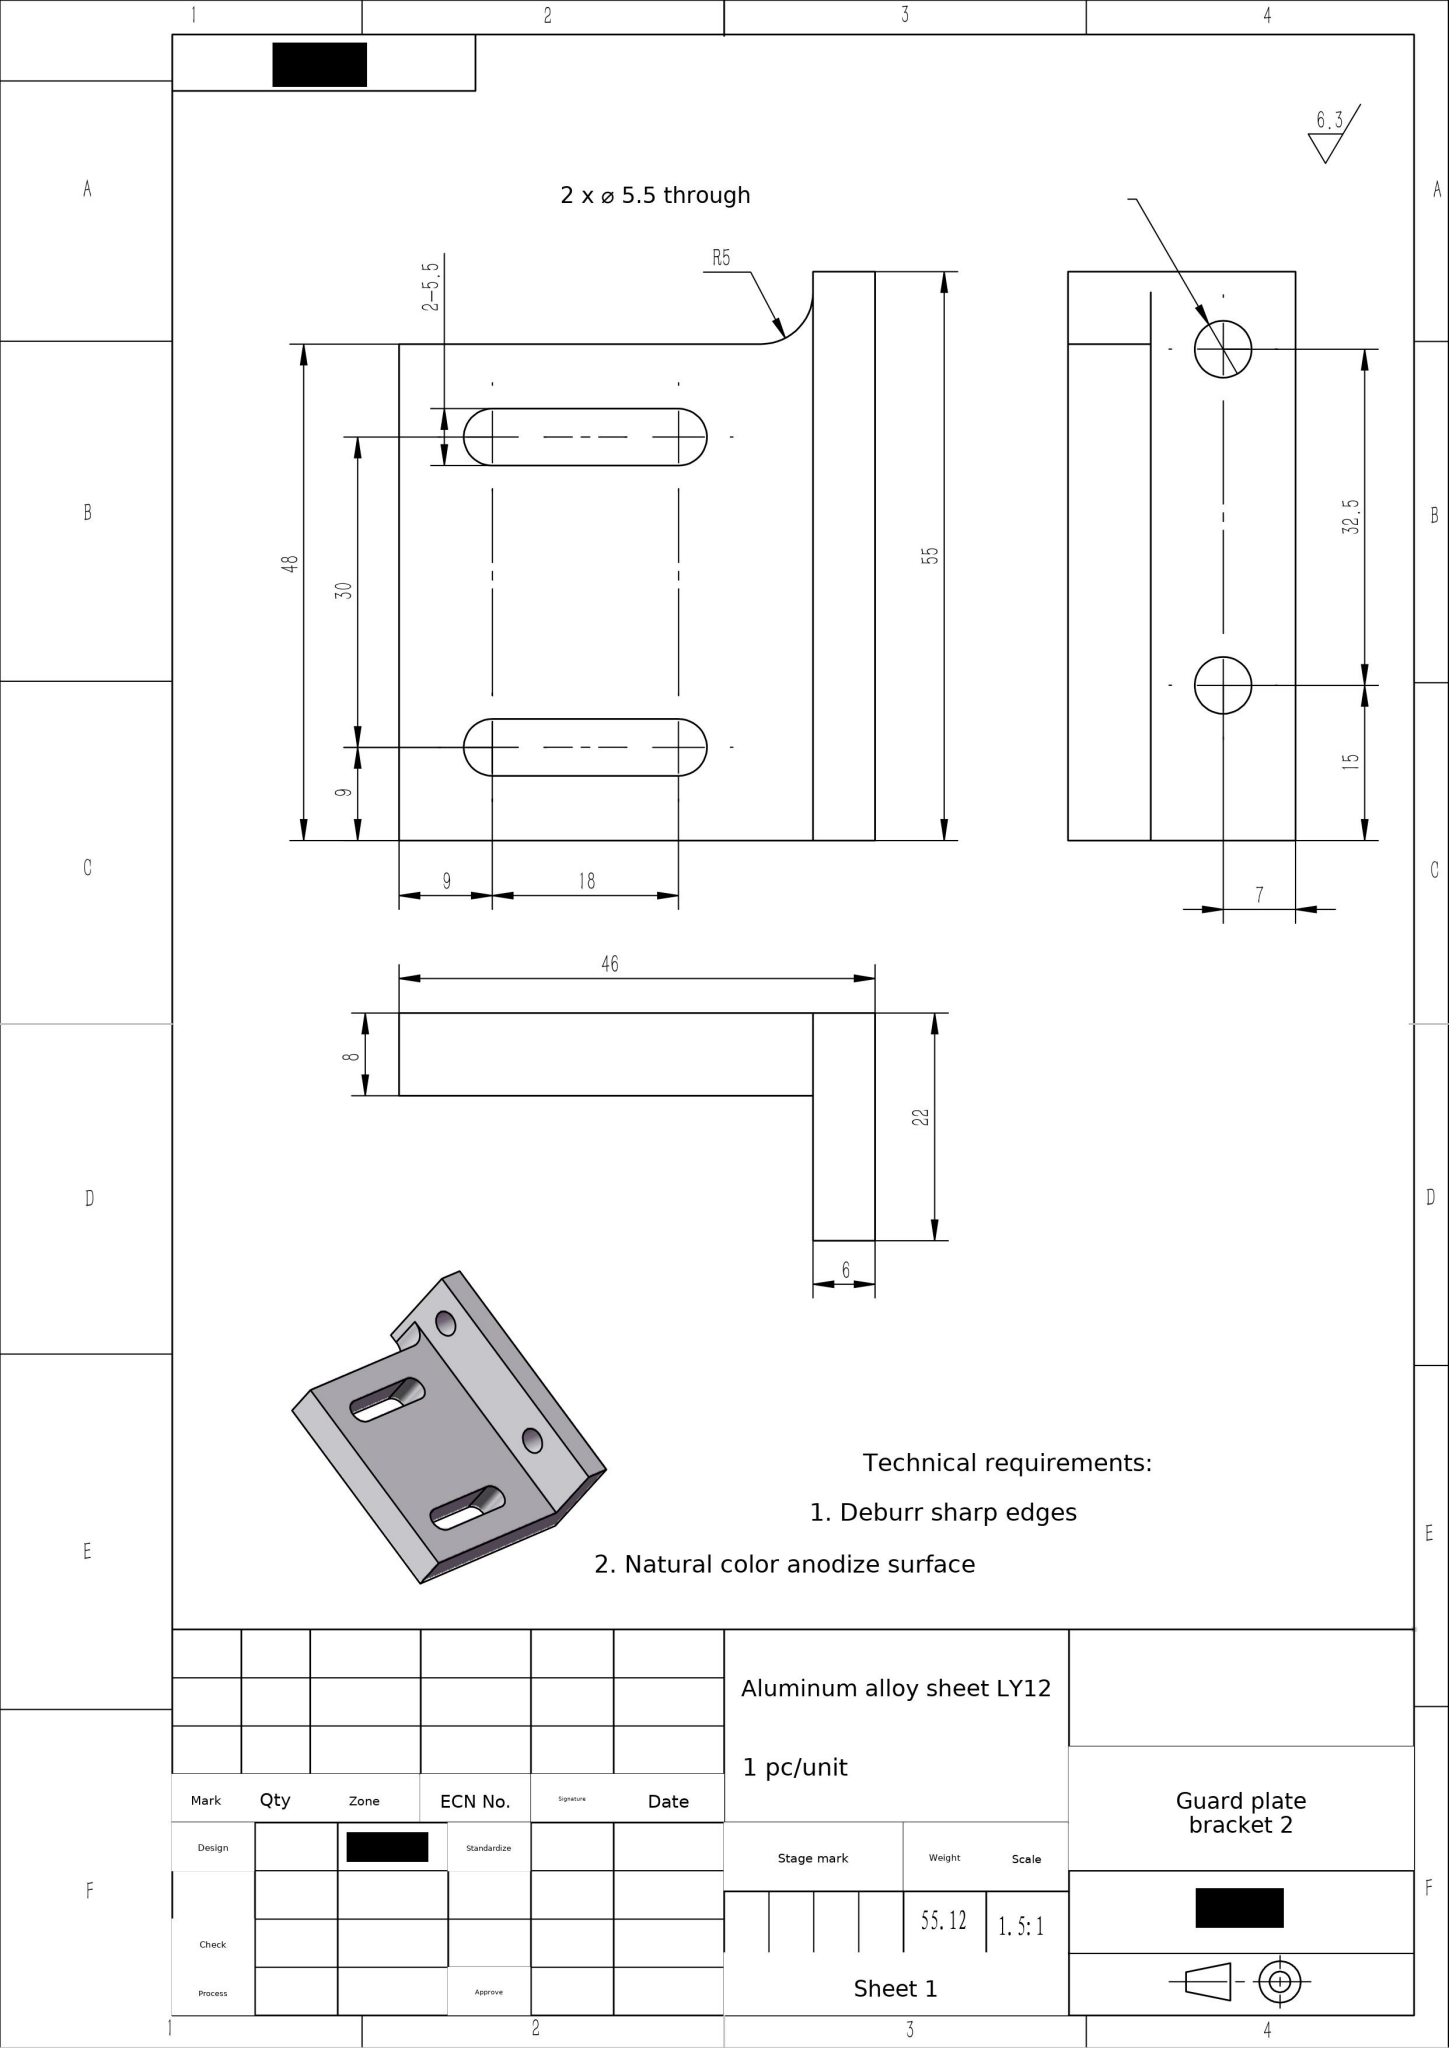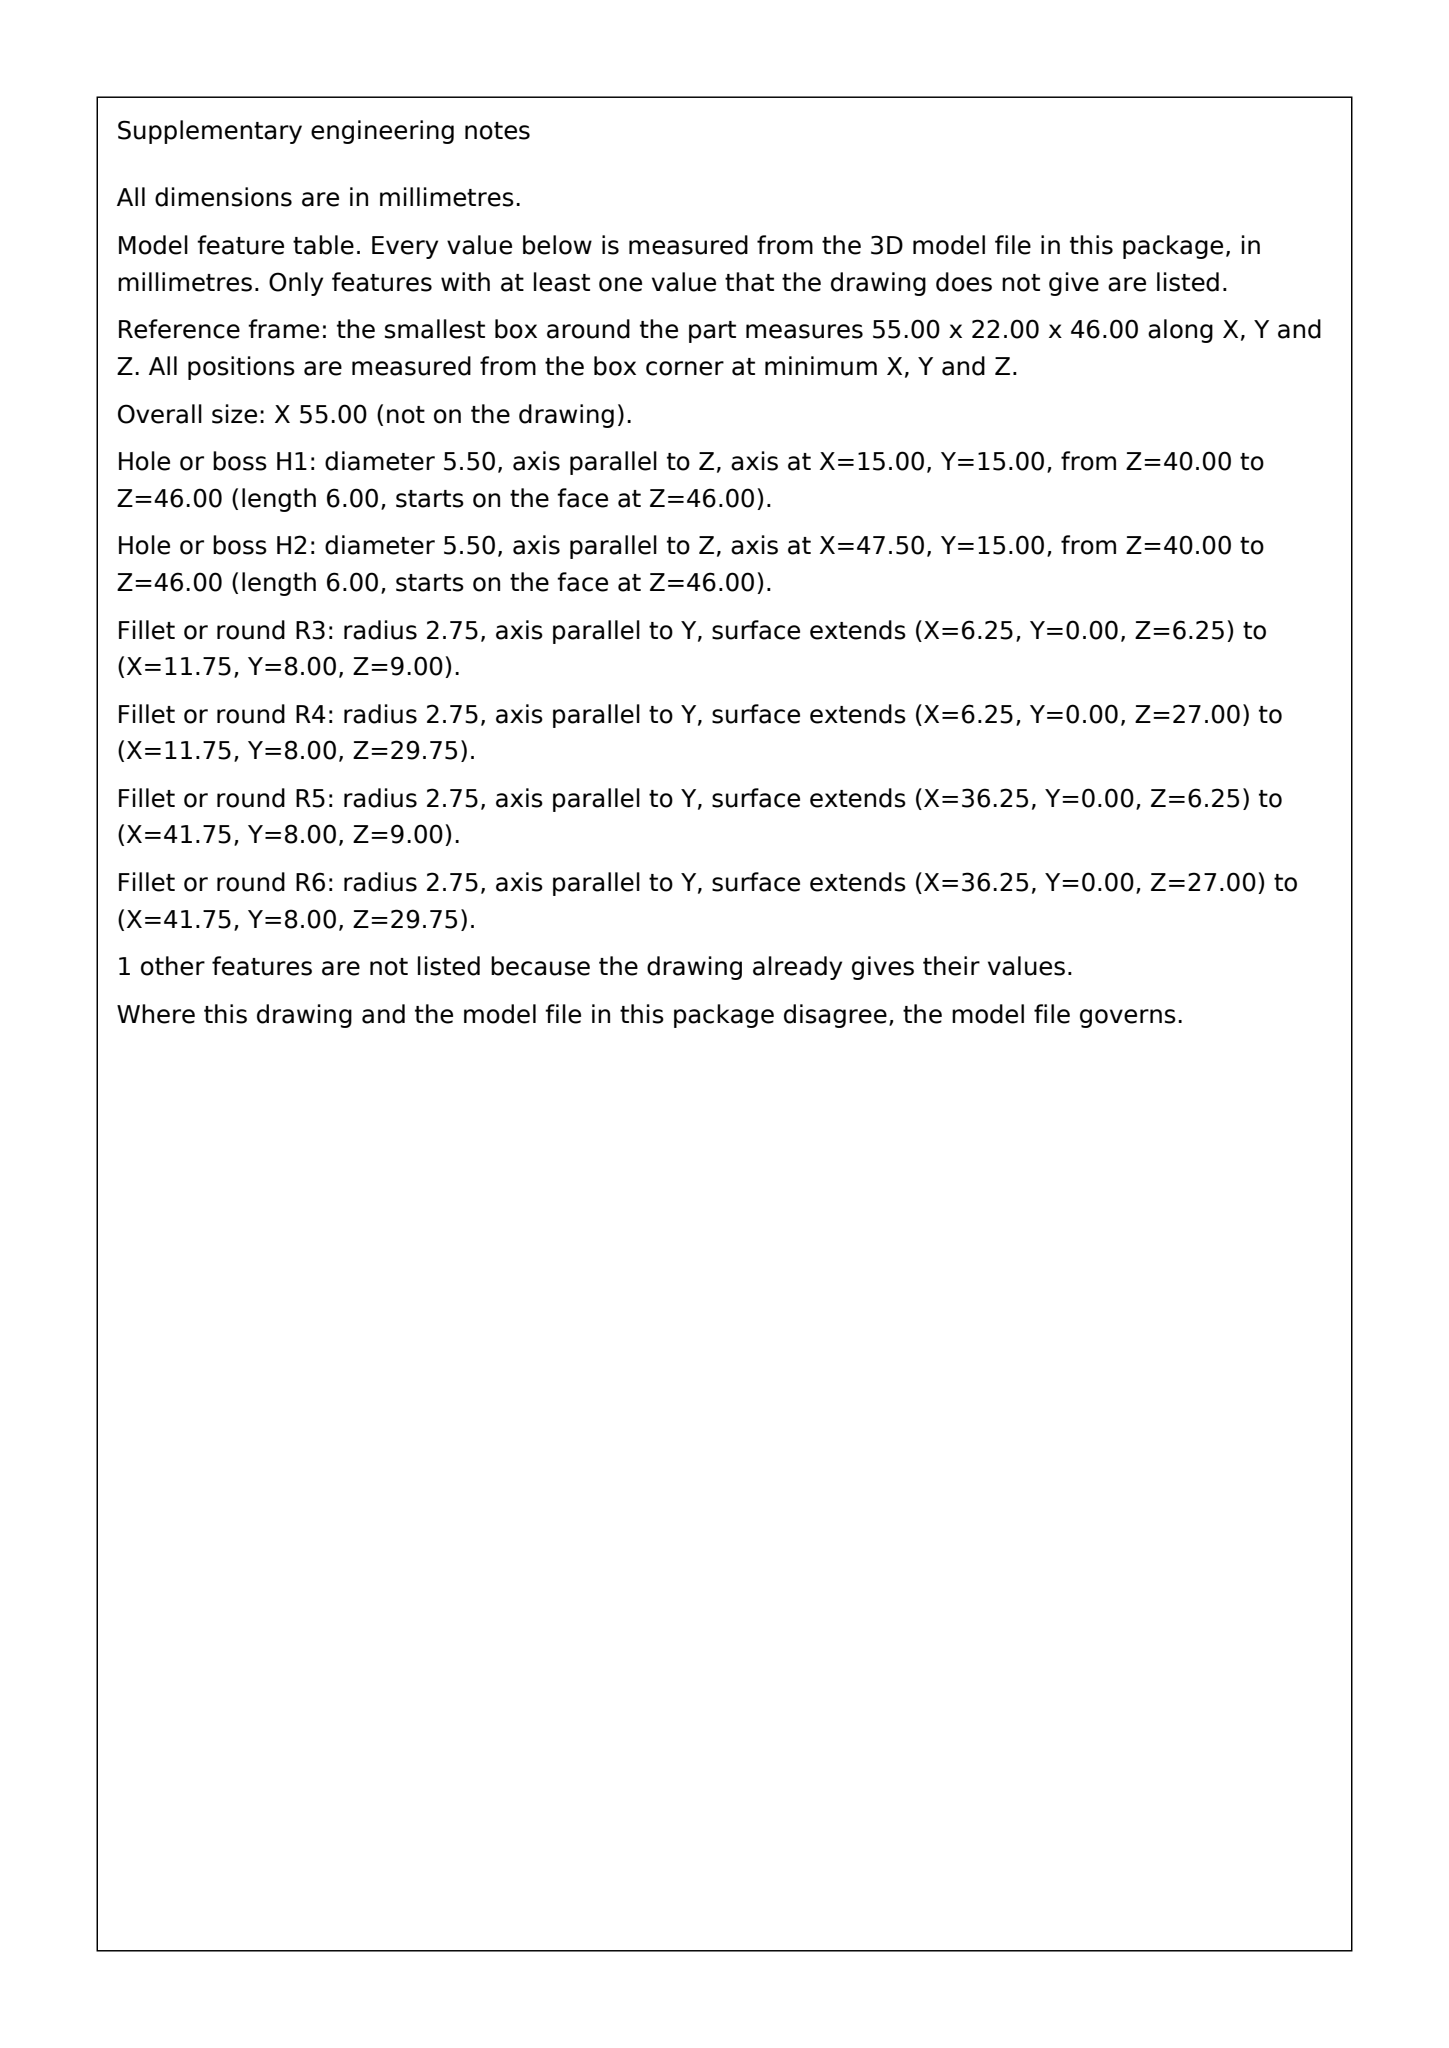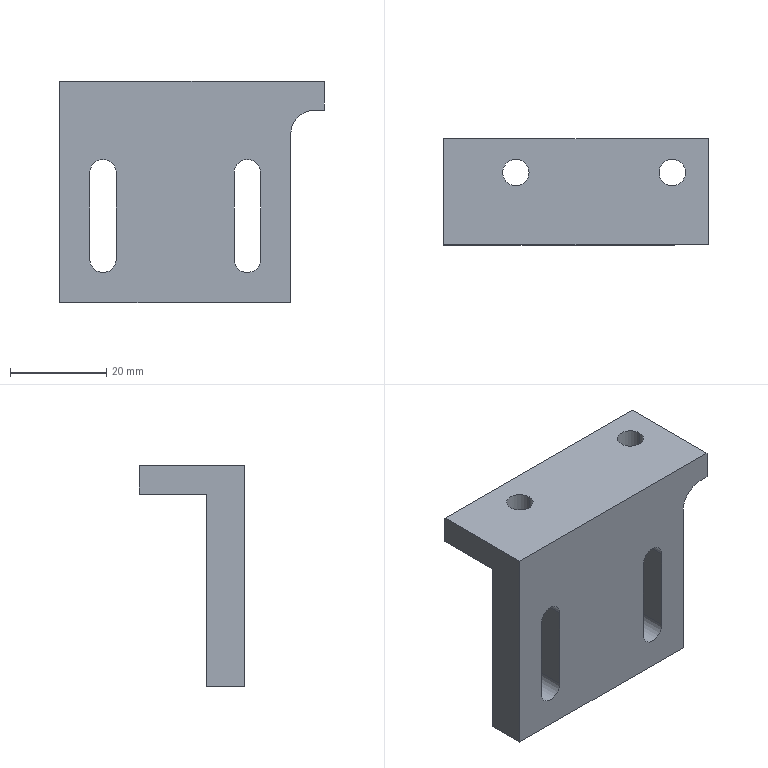Part | SolidWorks | mm | material Aluminum alloy sheet LY12 | 1 solid | 24 faces | box 55 x 22 x 46 mm | volume 20414 mm3 | plane 13 | cylinder 11 | commonest cylinder face diameters 5.5 x10 10 x1
build123d program:
from build123d import *

# Parameters (mm, degrees)
BOSS_EXTRUDE1_DEPTH            = 27.5
CUT_EXTRUDE1_DEPTH             = 72.723
SKETCH4_W                      = 55
SKETCH4_H                      = 14
BOSS_EXTRUDE2_DEPTH            = 6
F_5_5_5_5_DIAMETER_HOLE2_D     = 5.5
F_5_5_5_5_DIAMETER_HOLE2_DEPTH = 6
SKETCH7_W                      = 7
SKETCH7_H                      = 30
CUT_EXTRUDE2_DEPTH             = 79.334
SKETCH8_W                      = 55
SKETCH8_H                      = 30
CUT_EXTRUDE3_DEPTH             = 79.334
MOVE_FACE1_BY                  = 10
CUT_EXTRUDE4_DEPTH             = 73.858
SKETCH10_W                     = 7
SKETCH10_H                     = 40
CUT_EXTRUDE5_DEPTH             = 73.858
FILLET1_R                      = 5


with BuildPart() as part:
    # Sketch2 → Boss-Extrude1 (new, symmetric)
    with BuildSketch(Plane(origin=(0, 0, 0), x_dir=(0, 0, -1), z_dir=(1, 0, 0))):
        Polygon((0, 0), (0, 32), (-8, 32), (-8, 8), (-66, 8), (-66, 0), align=None)
    extrude(amount=BOSS_EXTRUDE1_DEPTH, both=True)

    # Sketch3 → Cut-Extrude1 (cut, through all)
    with BuildSketch(Plane.XY.offset(8)):
        with BuildLine():
            Line((8, 25.25), (16, 25.25))
            ThreePointArc((16, 25.25), (19.25, 22), (16, 18.75))
            Line((16, 18.75), (8, 18.75))
            ThreePointArc((8, 18.75), (4.75, 22), (8, 25.25))
        make_face()
        with BuildLine():
            Line((-18, 25.25), (-10, 25.25))
            ThreePointArc((-10, 25.25), (-6.75, 22), (-10, 18.75))
            Line((-10, 18.75), (-18, 18.75))
            ThreePointArc((-18, 18.75), (-21.25, 22), (-18, 25.25))
        make_face()
    extrude(amount=-CUT_EXTRUDE1_DEPTH, mode=Mode.SUBTRACT)

    # Sketch4 → Boss-Extrude2 (add)
    with BuildSketch(Plane.XY.offset(66)):
        with Locations((0, 15)):
            Rectangle(SKETCH4_W, SKETCH4_H)
    extrude(amount=-BOSS_EXTRUDE2_DEPTH)

    # 5.5 _5.5_ Diameter Hole2
    with Locations(Plane.XY.offset(66)):
        with Locations((-12.5, 15), (20, 15)):
            Hole(F_5_5_5_5_DIAMETER_HOLE2_D / 2, depth=F_5_5_5_5_DIAMETER_HOLE2_DEPTH)

    # Sketch7 → Cut-Extrude2 (cut, through all)
    with BuildSketch(Plane(origin=(0, 32, 0), x_dir=(1, 0, 0), z_dir=(0, 1, 0))):
        with Locations((24, -15)):
            Rectangle(SKETCH7_W, SKETCH7_H)
    extrude(amount=-CUT_EXTRUDE2_DEPTH, mode=Mode.SUBTRACT)

    # Sketch8 → Cut-Extrude3 (cut, through all)
    with BuildSketch(Plane(origin=(0, 32, 0), x_dir=(1, 0, 0), z_dir=(0, 1, 0))):
        with Locations((0, -15)):
            Rectangle(SKETCH8_W, SKETCH8_H)
    extrude(amount=-CUT_EXTRUDE3_DEPTH, mode=Mode.SUBTRACT)

    # Move Face1: a face moved outward by 10.0
    extrude(part.faces().sort_by_distance((0, 4, 30))[0], amount=MOVE_FACE1_BY, dir=(0, 0, -1))

    # Sketch9 → Cut-Extrude4 (cut, through all)
    with BuildSketch(Plane(origin=(0, 8, 0), x_dir=(1, 0, 0), z_dir=(0, 1, 0))):
        with BuildLine():
            Line((-15.75, -29), (-15.75, -47))
            ThreePointArc((-15.75, -47), (-18.5, -49.75), (-21.25, -47))
            Line((-21.25, -47), (-21.25, -29))
            ThreePointArc((-21.25, -29), (-18.5, -26.25), (-15.75, -29))
        make_face()
        with BuildLine():
            Line((14.25, -29), (14.25, -47))
            ThreePointArc((14.25, -47), (11.5, -49.75), (8.75, -47))
            Line((8.75, -47), (8.75, -29))
            ThreePointArc((8.75, -29), (11.5, -26.25), (14.25, -29))
        make_face()
    extrude(amount=-CUT_EXTRUDE4_DEPTH, mode=Mode.SUBTRACT)

    # Sketch10 → Cut-Extrude5 (cut, through all)
    with BuildSketch(Plane(origin=(0, 8, 0), x_dir=(1, 0, 0), z_dir=(0, 1, 0))):
        with Locations((24, -40)):
            Rectangle(SKETCH10_W, SKETCH10_H)
    extrude(amount=-CUT_EXTRUDE5_DEPTH, mode=Mode.SUBTRACT)

    # Fillet1
    fillet1_edges = [part.edges().sort_by_distance(p)[0] for p in [
        (20.5, 4, 60),
    ]]
    fillet(fillet1_edges, radius=FILLET1_R)


solid = part.part
STEP:
#1=CARTESIAN_POINT('',(-18.5,-0.,49.75));
#2=VERTEX_POINT('',#1);
#3=CARTESIAN_POINT('',(-15.75,-0.,47.));
#4=VERTEX_POINT('',#3);
#5=CARTESIAN_POINT('',(-18.5,-0.,47.));
#6=DIRECTION('',(0.,1.,0.));
#7=DIRECTION('',(0.,-0.,1.));
#8=AXIS2_PLACEMENT_3D('',#5,#6,#7);
#9=CIRCLE('',#8,2.75);
#10=EDGE_CURVE('',#2,#4,#9,.T.);
#11=ORIENTED_EDGE('',*,*,#10,.F.);
#12=CARTESIAN_POINT('',(-18.5,8.,49.75));
#13=VERTEX_POINT('',#12);
#14=CARTESIAN_POINT('',(-18.5,-0.,49.75));
#15=DIRECTION('',(0.,1.,0.));
#16=VECTOR('',#15,1000.);
#17=LINE('',#14,#16);
#18=EDGE_CURVE('',#2,#13,#17,.T.);
#19=ORIENTED_EDGE('',*,*,#18,.T.);
#20=CARTESIAN_POINT('',(-15.75,8.,47.));
#21=VERTEX_POINT('',#20);
#22=CARTESIAN_POINT('',(-18.5,8.,47.));
#23=DIRECTION('',(0.,1.,0.));
#24=DIRECTION('',(0.,0.,1.));
#25=AXIS2_PLACEMENT_3D('',#22,#23,#24);
#26=CIRCLE('',#25,2.75);
#27=EDGE_CURVE('',#13,#21,#26,.T.);
#28=ORIENTED_EDGE('',*,*,#27,.T.);
#29=CARTESIAN_POINT('',(-15.75,-0.,47.));
#30=DIRECTION('',(0.,1.,0.));
#31=VECTOR('',#30,1000.);
#32=LINE('',#29,#31);
#33=EDGE_CURVE('',#4,#21,#32,.T.);
#34=ORIENTED_EDGE('',*,*,#33,.F.);
#35=EDGE_LOOP('',(#11,#19,#28,#34));
#36=FACE_OUTER_BOUND('',#35,.T.);
#37=CARTESIAN_POINT('',(-18.5,-0.,47.));
#38=DIRECTION('',(0.,1.,0.));
#39=DIRECTION('',(0.,-0.,1.));
#40=AXIS2_PLACEMENT_3D('',#37,#38,#39);
#41=CYLINDRICAL_SURFACE('',#40,2.75);
#42=ADVANCED_FACE('',(#36),#41,.F.);
#43=CARTESIAN_POINT('',(11.5,-0.,49.75));
#44=VERTEX_POINT('',#43);
#45=CARTESIAN_POINT('',(14.25,-0.,47.));
#46=VERTEX_POINT('',#45);
#47=CARTESIAN_POINT('',(11.5,-0.,47.));
#48=DIRECTION('',(0.,1.,0.));
#49=DIRECTION('',(0.,-0.,1.));
#50=AXIS2_PLACEMENT_3D('',#47,#48,#49);
#51=CIRCLE('',#50,2.75);
#52=EDGE_CURVE('',#44,#46,#51,.T.);
#53=ORIENTED_EDGE('',*,*,#52,.F.);
#54=CARTESIAN_POINT('',(11.5,8.,49.75));
#55=VERTEX_POINT('',#54);
#56=CARTESIAN_POINT('',(11.5,-0.,49.75));
#57=DIRECTION('',(0.,1.,0.));
#58=VECTOR('',#57,1000.);
#59=LINE('',#56,#58);
#60=EDGE_CURVE('',#44,#55,#59,.T.);
#61=ORIENTED_EDGE('',*,*,#60,.T.);
#62=CARTESIAN_POINT('',(14.25,8.,47.));
#63=VERTEX_POINT('',#62);
#64=CARTESIAN_POINT('',(11.5,8.,47.));
#65=DIRECTION('',(0.,1.,0.));
#66=DIRECTION('',(0.,0.,1.));
#67=AXIS2_PLACEMENT_3D('',#64,#65,#66);
#68=CIRCLE('',#67,2.75);
#69=EDGE_CURVE('',#55,#63,#68,.T.);
#70=ORIENTED_EDGE('',*,*,#69,.T.);
#71=CARTESIAN_POINT('',(14.25,-0.,47.));
#72=DIRECTION('',(0.,1.,0.));
#73=VECTOR('',#72,1000.);
#74=LINE('',#71,#73);
#75=EDGE_CURVE('',#46,#63,#74,.T.);
#76=ORIENTED_EDGE('',*,*,#75,.F.);
#77=EDGE_LOOP('',(#53,#61,#70,#76));
#78=FACE_OUTER_BOUND('',#77,.T.);
#79=CARTESIAN_POINT('',(11.5,-0.,47.));
#80=DIRECTION('',(0.,1.,0.));
#81=DIRECTION('',(0.,-0.,1.));
#82=AXIS2_PLACEMENT_3D('',#79,#80,#81);
#83=CYLINDRICAL_SURFACE('',#82,2.75);
#84=ADVANCED_FACE('',(#78),#83,.F.);
#85=CARTESIAN_POINT('',(-9.75,15.,60.));
#86=VERTEX_POINT('',#85);
#87=CARTESIAN_POINT('',(-15.25,15.,60.));
#88=VERTEX_POINT('',#87);
#89=CARTESIAN_POINT('',(-12.5,15.,60.));
#90=DIRECTION('',(0.,0.,-1.));
#91=DIRECTION('',(-1.,0.,0.));
#92=AXIS2_PLACEMENT_3D('',#89,#90,#91);
#93=CIRCLE('',#92,2.75);
#94=EDGE_CURVE('',#86,#88,#93,.T.);
#95=ORIENTED_EDGE('',*,*,#94,.T.);
#96=CARTESIAN_POINT('',(-15.25,15.,66.));
#97=VERTEX_POINT('',#96);
#98=CARTESIAN_POINT('',(-15.25,15.,66.));
#99=DIRECTION('',(0.,0.,1.));
#100=VECTOR('',#99,1000.);
#101=LINE('',#98,#100);
#102=EDGE_CURVE('',#88,#97,#101,.T.);
#103=ORIENTED_EDGE('',*,*,#102,.T.);
#104=CARTESIAN_POINT('',(-9.75,15.,66.));
#105=VERTEX_POINT('',#104);
#106=CARTESIAN_POINT('',(-12.5,15.,66.));
#107=DIRECTION('',(0.,0.,1.));
#108=DIRECTION('',(1.,0.,0.));
#109=AXIS2_PLACEMENT_3D('',#106,#107,#108);
#110=CIRCLE('',#109,2.75);
#111=EDGE_CURVE('',#97,#105,#110,.T.);
#112=ORIENTED_EDGE('',*,*,#111,.T.);
#113=CARTESIAN_POINT('',(-9.75,15.,66.));
#114=DIRECTION('',(0.,0.,1.));
#115=VECTOR('',#114,1000.);
#116=LINE('',#113,#115);
#117=EDGE_CURVE('',#86,#105,#116,.T.);
#118=ORIENTED_EDGE('',*,*,#117,.F.);
#119=EDGE_LOOP('',(#95,#103,#112,#118));
#120=FACE_OUTER_BOUND('',#119,.T.);
#121=CARTESIAN_POINT('',(-12.5,15.,66.));
#122=DIRECTION('',(0.,0.,1.));
#123=DIRECTION('',(1.,0.,0.));
#124=AXIS2_PLACEMENT_3D('',#121,#122,#123);
#125=CYLINDRICAL_SURFACE('',#124,2.75);
#126=ADVANCED_FACE('',(#120),#125,.F.);
#127=CARTESIAN_POINT('',(22.75,15.,60.));
#128=VERTEX_POINT('',#127);
#129=CARTESIAN_POINT('',(17.25,15.,60.));
#130=VERTEX_POINT('',#129);
#131=CARTESIAN_POINT('',(20.,15.,60.));
#132=DIRECTION('',(0.,0.,-1.));
#133=DIRECTION('',(-1.,0.,0.));
#134=AXIS2_PLACEMENT_3D('',#131,#132,#133);
#135=CIRCLE('',#134,2.75);
#136=EDGE_CURVE('',#128,#130,#135,.T.);
#137=ORIENTED_EDGE('',*,*,#136,.T.);
#138=CARTESIAN_POINT('',(17.25,15.,66.));
#139=VERTEX_POINT('',#138);
#140=CARTESIAN_POINT('',(17.25,15.,66.));
#141=DIRECTION('',(0.,0.,1.));
#142=VECTOR('',#141,1000.);
#143=LINE('',#140,#142);
#144=EDGE_CURVE('',#130,#139,#143,.T.);
#145=ORIENTED_EDGE('',*,*,#144,.T.);
#146=CARTESIAN_POINT('',(22.75,15.,66.));
#147=VERTEX_POINT('',#146);
#148=CARTESIAN_POINT('',(20.,15.,66.));
#149=DIRECTION('',(0.,0.,1.));
#150=DIRECTION('',(1.,0.,0.));
#151=AXIS2_PLACEMENT_3D('',#148,#149,#150);
#152=CIRCLE('',#151,2.75);
#153=EDGE_CURVE('',#139,#147,#152,.T.);
#154=ORIENTED_EDGE('',*,*,#153,.T.);
#155=CARTESIAN_POINT('',(22.75,15.,66.));
#156=DIRECTION('',(0.,0.,1.));
#157=VECTOR('',#156,1000.);
#158=LINE('',#155,#157);
#159=EDGE_CURVE('',#128,#147,#158,.T.);
#160=ORIENTED_EDGE('',*,*,#159,.F.);
#161=EDGE_LOOP('',(#137,#145,#154,#160));
#162=FACE_OUTER_BOUND('',#161,.T.);
#163=CARTESIAN_POINT('',(20.,15.,66.));
#164=DIRECTION('',(0.,0.,1.));
#165=DIRECTION('',(1.,0.,0.));
#166=AXIS2_PLACEMENT_3D('',#163,#164,#165);
#167=CYLINDRICAL_SURFACE('',#166,2.75);
#168=ADVANCED_FACE('',(#162),#167,.F.);
#169=CARTESIAN_POINT('',(-15.75,-0.,29.));
#170=VERTEX_POINT('',#169);
#171=CARTESIAN_POINT('',(-15.75,-0.,29.));
#172=DIRECTION('',(-0.,0.,-1.));
#173=VECTOR('',#172,1000.);
#174=LINE('',#171,#173);
#175=EDGE_CURVE('',#4,#170,#174,.T.);
#176=ORIENTED_EDGE('',*,*,#175,.T.);
#177=CARTESIAN_POINT('',(-21.25,-0.,29.));
#178=VERTEX_POINT('',#177);
#179=CARTESIAN_POINT('',(-18.5,-0.,29.));
#180=DIRECTION('',(0.,1.,0.));
#181=DIRECTION('',(0.,-0.,1.));
#182=AXIS2_PLACEMENT_3D('',#179,#180,#181);
#183=CIRCLE('',#182,2.75);
#184=EDGE_CURVE('',#170,#178,#183,.T.);
#185=ORIENTED_EDGE('',*,*,#184,.T.);
#186=CARTESIAN_POINT('',(-21.25,0.,47.));
#187=VERTEX_POINT('',#186);
#188=CARTESIAN_POINT('',(-21.25,-0.,29.));
#189=DIRECTION('',(0.,0.,1.));
#190=VECTOR('',#189,1000.);
#191=LINE('',#188,#190);
#192=EDGE_CURVE('',#178,#187,#191,.T.);
#193=ORIENTED_EDGE('',*,*,#192,.T.);
#194=CARTESIAN_POINT('',(-18.5,-0.,47.));
#195=DIRECTION('',(0.,1.,0.));
#196=DIRECTION('',(0.,-0.,1.));
#197=AXIS2_PLACEMENT_3D('',#194,#195,#196);
#198=CIRCLE('',#197,2.75);
#199=EDGE_CURVE('',#187,#2,#198,.T.);
#200=ORIENTED_EDGE('',*,*,#199,.T.);
#201=ORIENTED_EDGE('',*,*,#10,.T.);
#202=EDGE_LOOP('',(#176,#185,#193,#200,#201));
#203=FACE_BOUND('',#202,.T.);
#204=CARTESIAN_POINT('',(14.25,0.,29.));
#205=VERTEX_POINT('',#204);
#206=CARTESIAN_POINT('',(14.25,0.,29.));
#207=DIRECTION('',(0.,0.,-1.));
#208=VECTOR('',#207,1000.);
#209=LINE('',#206,#208);
#210=EDGE_CURVE('',#46,#205,#209,.T.);
#211=ORIENTED_EDGE('',*,*,#210,.T.);
#212=CARTESIAN_POINT('',(8.75,0.,29.));
#213=VERTEX_POINT('',#212);
#214=CARTESIAN_POINT('',(11.5,-0.,29.));
#215=DIRECTION('',(0.,1.,0.));
#216=DIRECTION('',(0.,-0.,1.));
#217=AXIS2_PLACEMENT_3D('',#214,#215,#216);
#218=CIRCLE('',#217,2.75);
#219=EDGE_CURVE('',#205,#213,#218,.T.);
#220=ORIENTED_EDGE('',*,*,#219,.T.);
#221=CARTESIAN_POINT('',(8.75,0.,47.));
#222=VERTEX_POINT('',#221);
#223=CARTESIAN_POINT('',(8.75,0.,29.));
#224=DIRECTION('',(-0.,-0.,1.));
#225=VECTOR('',#224,1000.);
#226=LINE('',#223,#225);
#227=EDGE_CURVE('',#213,#222,#226,.T.);
#228=ORIENTED_EDGE('',*,*,#227,.T.);
#229=CARTESIAN_POINT('',(11.5,-0.,47.));
#230=DIRECTION('',(0.,1.,0.));
#231=DIRECTION('',(0.,-0.,1.));
#232=AXIS2_PLACEMENT_3D('',#229,#230,#231);
#233=CIRCLE('',#232,2.75);
#234=EDGE_CURVE('',#222,#44,#233,.T.);
#235=ORIENTED_EDGE('',*,*,#234,.T.);
#236=ORIENTED_EDGE('',*,*,#52,.T.);
#237=EDGE_LOOP('',(#211,#220,#228,#235,#236));
#238=FACE_BOUND('',#237,.T.);
#239=CARTESIAN_POINT('',(20.5,0.,20.));
#240=VERTEX_POINT('',#239);
#241=CARTESIAN_POINT('',(20.5,-0.,55.));
#242=VERTEX_POINT('',#241);
#243=CARTESIAN_POINT('',(20.5,-0.,20.));
#244=DIRECTION('',(0.,-0.,1.));
#245=VECTOR('',#244,1000.);
#246=LINE('',#243,#245);
#247=EDGE_CURVE('',#240,#242,#246,.T.);
#248=ORIENTED_EDGE('',*,*,#247,.T.);
#249=CARTESIAN_POINT('',(25.5,-0.,60.));
#250=VERTEX_POINT('',#249);
#251=CARTESIAN_POINT('',(25.5,0.,55.));
#252=DIRECTION('',(0.,1.,0.));
#253=DIRECTION('',(0.,0.,1.));
#254=AXIS2_PLACEMENT_3D('',#251,#252,#253);
#255=CIRCLE('',#254,5.);
#256=EDGE_CURVE('',#242,#250,#255,.T.);
#257=ORIENTED_EDGE('',*,*,#256,.T.);
#258=CARTESIAN_POINT('',(27.5,-0.,60.));
#259=VERTEX_POINT('',#258);
#260=CARTESIAN_POINT('',(27.5,-0.,60.));
#261=DIRECTION('',(1.,0.,0.));
#262=VECTOR('',#261,1000.);
#263=LINE('',#260,#262);
#264=EDGE_CURVE('',#250,#259,#263,.T.);
#265=ORIENTED_EDGE('',*,*,#264,.T.);
#266=CARTESIAN_POINT('',(27.5,0.,66.));
#267=VERTEX_POINT('',#266);
#268=CARTESIAN_POINT('',(27.5,0.,66.));
#269=DIRECTION('',(0.,0.,-1.));
#270=VECTOR('',#269,1000.);
#271=LINE('',#268,#270);
#272=EDGE_CURVE('',#267,#259,#271,.T.);
#273=ORIENTED_EDGE('',*,*,#272,.F.);
#274=CARTESIAN_POINT('',(-27.5,0.,66.));
#275=VERTEX_POINT('',#274);
#276=CARTESIAN_POINT('',(27.5,0.,66.));
#277=DIRECTION('',(-1.,0.,0.));
#278=VECTOR('',#277,1000.);
#279=LINE('',#276,#278);
#280=EDGE_CURVE('',#267,#275,#279,.T.);
#281=ORIENTED_EDGE('',*,*,#280,.T.);
#282=CARTESIAN_POINT('',(-27.5,0.,20.));
#283=VERTEX_POINT('',#282);
#284=CARTESIAN_POINT('',(-27.5,0.,66.));
#285=DIRECTION('',(0.,0.,-1.));
#286=VECTOR('',#285,1000.);
#287=LINE('',#284,#286);
#288=EDGE_CURVE('',#275,#283,#287,.T.);
#289=ORIENTED_EDGE('',*,*,#288,.T.);
#290=CARTESIAN_POINT('',(20.5,0.,20.));
#291=DIRECTION('',(1.,0.,0.));
#292=VECTOR('',#291,1000.);
#293=LINE('',#290,#292);
#294=EDGE_CURVE('',#283,#240,#293,.T.);
#295=ORIENTED_EDGE('',*,*,#294,.T.);
#296=EDGE_LOOP('',(#248,#257,#265,#273,#281,#289,#295));
#297=FACE_OUTER_BOUND('',#296,.T.);
#298=CARTESIAN_POINT('',(27.5,0.,66.));
#299=DIRECTION('',(0.,1.,0.));
#300=DIRECTION('',(0.,0.,1.));
#301=AXIS2_PLACEMENT_3D('',#298,#299,#300);
#302=PLANE('',#301);
#303=ADVANCED_FACE('',(#203,#238,#297),#302,.F.);
#304=CARTESIAN_POINT('',(-21.25,8.,29.));
#305=VERTEX_POINT('',#304);
#306=CARTESIAN_POINT('',(-21.25,8.,47.));
#307=VERTEX_POINT('',#306);
#308=CARTESIAN_POINT('',(-21.25,8.,29.));
#309=DIRECTION('',(0.,0.,1.));
#310=VECTOR('',#309,1000.);
#311=LINE('',#308,#310);
#312=EDGE_CURVE('',#305,#307,#311,.T.);
#313=ORIENTED_EDGE('',*,*,#312,.F.);
#314=CARTESIAN_POINT('',(-15.75,8.,29.));
#315=VERTEX_POINT('',#314);
#316=CARTESIAN_POINT('',(-18.5,8.,29.));
#317=DIRECTION('',(0.,1.,0.));
#318=DIRECTION('',(0.,0.,1.));
#319=AXIS2_PLACEMENT_3D('',#316,#317,#318);
#320=CIRCLE('',#319,2.75);
#321=EDGE_CURVE('',#315,#305,#320,.T.);
#322=ORIENTED_EDGE('',*,*,#321,.F.);
#323=CARTESIAN_POINT('',(-15.75,8.,29.));
#324=DIRECTION('',(-0.,0.,-1.));
#325=VECTOR('',#324,1000.);
#326=LINE('',#323,#325);
#327=EDGE_CURVE('',#21,#315,#326,.T.);
#328=ORIENTED_EDGE('',*,*,#327,.F.);
#329=ORIENTED_EDGE('',*,*,#27,.F.);
#330=CARTESIAN_POINT('',(-18.5,8.,47.));
#331=DIRECTION('',(0.,1.,0.));
#332=DIRECTION('',(0.,0.,1.));
#333=AXIS2_PLACEMENT_3D('',#330,#331,#332);
#334=CIRCLE('',#333,2.75);
#335=EDGE_CURVE('',#307,#13,#334,.T.);
#336=ORIENTED_EDGE('',*,*,#335,.F.);
#337=EDGE_LOOP('',(#313,#322,#328,#329,#336));
#338=FACE_BOUND('',#337,.T.);
#339=CARTESIAN_POINT('',(8.75,8.,29.));
#340=VERTEX_POINT('',#339);
#341=CARTESIAN_POINT('',(8.75,8.,47.));
#342=VERTEX_POINT('',#341);
#343=CARTESIAN_POINT('',(8.75,8.,29.));
#344=DIRECTION('',(-0.,-0.,1.));
#345=VECTOR('',#344,1000.);
#346=LINE('',#343,#345);
#347=EDGE_CURVE('',#340,#342,#346,.T.);
#348=ORIENTED_EDGE('',*,*,#347,.F.);
#349=CARTESIAN_POINT('',(14.25,8.,29.));
#350=VERTEX_POINT('',#349);
#351=CARTESIAN_POINT('',(11.5,8.,29.));
#352=DIRECTION('',(0.,1.,0.));
#353=DIRECTION('',(0.,0.,1.));
#354=AXIS2_PLACEMENT_3D('',#351,#352,#353);
#355=CIRCLE('',#354,2.75);
#356=EDGE_CURVE('',#350,#340,#355,.T.);
#357=ORIENTED_EDGE('',*,*,#356,.F.);
#358=CARTESIAN_POINT('',(14.25,8.,29.));
#359=DIRECTION('',(0.,0.,-1.));
#360=VECTOR('',#359,1000.);
#361=LINE('',#358,#360);
#362=EDGE_CURVE('',#63,#350,#361,.T.);
#363=ORIENTED_EDGE('',*,*,#362,.F.);
#364=ORIENTED_EDGE('',*,*,#69,.F.);
#365=CARTESIAN_POINT('',(11.5,8.,47.));
#366=DIRECTION('',(0.,1.,0.));
#367=DIRECTION('',(0.,0.,1.));
#368=AXIS2_PLACEMENT_3D('',#365,#366,#367);
#369=CIRCLE('',#368,2.75);
#370=EDGE_CURVE('',#342,#55,#369,.T.);
#371=ORIENTED_EDGE('',*,*,#370,.F.);
#372=EDGE_LOOP('',(#348,#357,#363,#364,#371));
#373=FACE_BOUND('',#372,.T.);
#374=CARTESIAN_POINT('',(-27.5,8.,60.));
#375=VERTEX_POINT('',#374);
#376=CARTESIAN_POINT('',(25.5,8.,60.));
#377=VERTEX_POINT('',#376);
#378=CARTESIAN_POINT('',(-27.5,8.,60.));
#379=DIRECTION('',(1.,0.,0.));
#380=VECTOR('',#379,1000.);
#381=LINE('',#378,#380);
#382=EDGE_CURVE('',#375,#377,#381,.T.);
#383=ORIENTED_EDGE('',*,*,#382,.T.);
#384=CARTESIAN_POINT('',(20.5,8.,55.));
#385=VERTEX_POINT('',#384);
#386=CARTESIAN_POINT('',(25.5,8.,55.));
#387=DIRECTION('',(0.,-1.,-0.));
#388=DIRECTION('',(0.,0.,-1.));
#389=AXIS2_PLACEMENT_3D('',#386,#387,#388);
#390=CIRCLE('',#389,5.);
#391=EDGE_CURVE('',#377,#385,#390,.T.);
#392=ORIENTED_EDGE('',*,*,#391,.T.);
#393=CARTESIAN_POINT('',(20.5,8.,20.));
#394=VERTEX_POINT('',#393);
#395=CARTESIAN_POINT('',(20.5,8.,20.));
#396=DIRECTION('',(0.,-0.,1.));
#397=VECTOR('',#396,1000.);
#398=LINE('',#395,#397);
#399=EDGE_CURVE('',#394,#385,#398,.T.);
#400=ORIENTED_EDGE('',*,*,#399,.F.);
#401=CARTESIAN_POINT('',(-27.5,8.,20.));
#402=VERTEX_POINT('',#401);
#403=CARTESIAN_POINT('',(27.5,8.,20.));
#404=DIRECTION('',(-1.,0.,0.));
#405=VECTOR('',#404,1000.);
#406=LINE('',#403,#405);
#407=EDGE_CURVE('',#394,#402,#406,.T.);
#408=ORIENTED_EDGE('',*,*,#407,.T.);
#409=CARTESIAN_POINT('',(-27.5,8.,8.));
#410=DIRECTION('',(0.,-0.,1.));
#411=VECTOR('',#410,1000.);
#412=LINE('',#409,#411);
#413=EDGE_CURVE('',#402,#375,#412,.T.);
#414=ORIENTED_EDGE('',*,*,#413,.T.);
#415=EDGE_LOOP('',(#383,#392,#400,#408,#414));
#416=FACE_OUTER_BOUND('',#415,.T.);
#417=CARTESIAN_POINT('',(27.5,8.,8.));
#418=DIRECTION('',(0.,-1.,-0.));
#419=DIRECTION('',(0.,0.,-1.));
#420=AXIS2_PLACEMENT_3D('',#417,#418,#419);
#421=PLANE('',#420);
#422=ADVANCED_FACE('',(#338,#373,#416),#421,.F.);
#423=CARTESIAN_POINT('',(-12.5,15.,66.));
#424=DIRECTION('',(0.,0.,1.));
#425=DIRECTION('',(1.,0.,0.));
#426=AXIS2_PLACEMENT_3D('',#423,#424,#425);
#427=CIRCLE('',#426,2.75);
#428=EDGE_CURVE('',#105,#97,#427,.T.);
#429=ORIENTED_EDGE('',*,*,#428,.F.);
#430=ORIENTED_EDGE('',*,*,#111,.F.);
#431=EDGE_LOOP('',(#429,#430));
#432=FACE_BOUND('',#431,.T.);
#433=CARTESIAN_POINT('',(20.,15.,66.));
#434=DIRECTION('',(0.,0.,1.));
#435=DIRECTION('',(1.,0.,0.));
#436=AXIS2_PLACEMENT_3D('',#433,#434,#435);
#437=CIRCLE('',#436,2.75);
#438=EDGE_CURVE('',#147,#139,#437,.T.);
#439=ORIENTED_EDGE('',*,*,#438,.F.);
#440=ORIENTED_EDGE('',*,*,#153,.F.);
#441=EDGE_LOOP('',(#439,#440));
#442=FACE_BOUND('',#441,.T.);
#443=CARTESIAN_POINT('',(-27.5,22.,66.));
#444=VERTEX_POINT('',#443);
#445=CARTESIAN_POINT('',(-27.5,8.,66.));
#446=DIRECTION('',(0.,-1.,0.));
#447=VECTOR('',#446,1000.);
#448=LINE('',#445,#447);
#449=EDGE_CURVE('',#444,#275,#448,.T.);
#450=ORIENTED_EDGE('',*,*,#449,.T.);
#451=ORIENTED_EDGE('',*,*,#280,.F.);
#452=CARTESIAN_POINT('',(27.5,22.,66.));
#453=VERTEX_POINT('',#452);
#454=CARTESIAN_POINT('',(27.5,8.,66.));
#455=DIRECTION('',(0.,-1.,0.));
#456=VECTOR('',#455,1000.);
#457=LINE('',#454,#456);
#458=EDGE_CURVE('',#453,#267,#457,.T.);
#459=ORIENTED_EDGE('',*,*,#458,.F.);
#460=CARTESIAN_POINT('',(-27.5,22.,66.));
#461=DIRECTION('',(-1.,0.,0.));
#462=VECTOR('',#461,1000.);
#463=LINE('',#460,#462);
#464=EDGE_CURVE('',#453,#444,#463,.T.);
#465=ORIENTED_EDGE('',*,*,#464,.T.);
#466=EDGE_LOOP('',(#450,#451,#459,#465));
#467=FACE_OUTER_BOUND('',#466,.T.);
#468=CARTESIAN_POINT('',(27.5,8.,66.));
#469=DIRECTION('',(0.,0.,-1.));
#470=DIRECTION('',(-1.,0.,0.));
#471=AXIS2_PLACEMENT_3D('',#468,#469,#470);
#472=PLANE('',#471);
#473=ADVANCED_FACE('',(#432,#442,#467),#472,.F.);
#474=ORIENTED_EDGE('',*,*,#272,.T.);
#475=CARTESIAN_POINT('',(27.5,22.,60.));
#476=VERTEX_POINT('',#475);
#477=CARTESIAN_POINT('',(27.5,8.,60.));
#478=DIRECTION('',(0.,1.,0.));
#479=VECTOR('',#478,1000.);
#480=LINE('',#477,#479);
#481=EDGE_CURVE('',#259,#476,#480,.T.);
#482=ORIENTED_EDGE('',*,*,#481,.T.);
#483=CARTESIAN_POINT('',(27.5,22.,60.));
#484=DIRECTION('',(0.,0.,1.));
#485=VECTOR('',#484,1000.);
#486=LINE('',#483,#485);
#487=EDGE_CURVE('',#476,#453,#486,.T.);
#488=ORIENTED_EDGE('',*,*,#487,.T.);
#489=ORIENTED_EDGE('',*,*,#458,.T.);
#490=EDGE_LOOP('',(#474,#482,#488,#489));
#491=FACE_OUTER_BOUND('',#490,.T.);
#492=CARTESIAN_POINT('',(27.5,0.,0.));
#493=DIRECTION('',(1.,0.,0.));
#494=DIRECTION('',(0.,0.,-1.));
#495=AXIS2_PLACEMENT_3D('',#492,#493,#494);
#496=PLANE('',#495);
#497=ADVANCED_FACE('',(#491),#496,.T.);
#498=ORIENTED_EDGE('',*,*,#413,.F.);
#499=CARTESIAN_POINT('',(-27.5,0.,20.));
#500=DIRECTION('',(0.,1.,0.));
#501=VECTOR('',#500,1000.);
#502=LINE('',#499,#501);
#503=EDGE_CURVE('',#283,#402,#502,.T.);
#504=ORIENTED_EDGE('',*,*,#503,.F.);
#505=ORIENTED_EDGE('',*,*,#288,.F.);
#506=ORIENTED_EDGE('',*,*,#449,.F.);
#507=CARTESIAN_POINT('',(-27.5,22.,60.));
#508=VERTEX_POINT('',#507);
#509=CARTESIAN_POINT('',(-27.5,22.,60.));
#510=DIRECTION('',(0.,0.,1.));
#511=VECTOR('',#510,1000.);
#512=LINE('',#509,#511);
#513=EDGE_CURVE('',#508,#444,#512,.T.);
#514=ORIENTED_EDGE('',*,*,#513,.F.);
#515=CARTESIAN_POINT('',(-27.5,8.,60.));
#516=DIRECTION('',(0.,-1.,0.));
#517=VECTOR('',#516,1000.);
#518=LINE('',#515,#517);
#519=EDGE_CURVE('',#508,#375,#518,.T.);
#520=ORIENTED_EDGE('',*,*,#519,.T.);
#521=EDGE_LOOP('',(#498,#504,#505,#506,#514,#520));
#522=FACE_OUTER_BOUND('',#521,.T.);
#523=CARTESIAN_POINT('',(-27.5,0.,0.));
#524=DIRECTION('',(1.,0.,0.));
#525=DIRECTION('',(0.,0.,-1.));
#526=AXIS2_PLACEMENT_3D('',#523,#524,#525);
#527=PLANE('',#526);
#528=ADVANCED_FACE('',(#522),#527,.F.);
#529=ORIENTED_EDGE('',*,*,#464,.F.);
#530=ORIENTED_EDGE('',*,*,#487,.F.);
#531=CARTESIAN_POINT('',(-27.5,22.,60.));
#532=DIRECTION('',(-1.,0.,0.));
#533=VECTOR('',#532,1000.);
#534=LINE('',#531,#533);
#535=EDGE_CURVE('',#476,#508,#534,.T.);
#536=ORIENTED_EDGE('',*,*,#535,.T.);
#537=ORIENTED_EDGE('',*,*,#513,.T.);
#538=EDGE_LOOP('',(#529,#530,#536,#537));
#539=FACE_OUTER_BOUND('',#538,.T.);
#540=CARTESIAN_POINT('',(-27.5,22.,60.));
#541=DIRECTION('',(0.,1.,0.));
#542=DIRECTION('',(0.,0.,1.));
#543=AXIS2_PLACEMENT_3D('',#540,#541,#542);
#544=PLANE('',#543);
#545=ADVANCED_FACE('',(#539),#544,.T.);
#546=ORIENTED_EDGE('',*,*,#94,.F.);
#547=CARTESIAN_POINT('',(-12.5,15.,60.));
#548=DIRECTION('',(0.,0.,-1.));
#549=DIRECTION('',(-1.,0.,0.));
#550=AXIS2_PLACEMENT_3D('',#547,#548,#549);
#551=CIRCLE('',#550,2.75);
#552=EDGE_CURVE('',#88,#86,#551,.T.);
#553=ORIENTED_EDGE('',*,*,#552,.F.);
#554=EDGE_LOOP('',(#546,#553));
#555=FACE_BOUND('',#554,.T.);
#556=ORIENTED_EDGE('',*,*,#136,.F.);
#557=CARTESIAN_POINT('',(20.,15.,60.));
#558=DIRECTION('',(0.,0.,-1.));
#559=DIRECTION('',(-1.,0.,0.));
#560=AXIS2_PLACEMENT_3D('',#557,#558,#559);
#561=CIRCLE('',#560,2.75);
#562=EDGE_CURVE('',#130,#128,#561,.T.);
#563=ORIENTED_EDGE('',*,*,#562,.F.);
#564=EDGE_LOOP('',(#556,#563));
#565=FACE_BOUND('',#564,.T.);
#566=ORIENTED_EDGE('',*,*,#264,.F.);
#567=CARTESIAN_POINT('',(25.5,0.,60.));
#568=DIRECTION('',(-0.,1.,0.));
#569=VECTOR('',#568,1000.);
#570=LINE('',#567,#569);
#571=EDGE_CURVE('',#250,#377,#570,.T.);
#572=ORIENTED_EDGE('',*,*,#571,.T.);
#573=ORIENTED_EDGE('',*,*,#382,.F.);
#574=ORIENTED_EDGE('',*,*,#519,.F.);
#575=ORIENTED_EDGE('',*,*,#535,.F.);
#576=ORIENTED_EDGE('',*,*,#481,.F.);
#577=EDGE_LOOP('',(#566,#572,#573,#574,#575,#576));
#578=FACE_OUTER_BOUND('',#577,.T.);
#579=CARTESIAN_POINT('',(0.,0.,60.));
#580=DIRECTION('',(0.,0.,-1.));
#581=DIRECTION('',(-1.,0.,0.));
#582=AXIS2_PLACEMENT_3D('',#579,#580,#581);
#583=PLANE('',#582);
#584=ADVANCED_FACE('',(#555,#565,#578),#583,.T.);
#585=ORIENTED_EDGE('',*,*,#144,.F.);
#586=ORIENTED_EDGE('',*,*,#562,.T.);
#587=ORIENTED_EDGE('',*,*,#159,.T.);
#588=ORIENTED_EDGE('',*,*,#438,.T.);
#589=EDGE_LOOP('',(#585,#586,#587,#588));
#590=FACE_OUTER_BOUND('',#589,.T.);
#591=CARTESIAN_POINT('',(20.,15.,66.));
#592=DIRECTION('',(0.,0.,1.));
#593=DIRECTION('',(1.,0.,0.));
#594=AXIS2_PLACEMENT_3D('',#591,#592,#593);
#595=CYLINDRICAL_SURFACE('',#594,2.75);
#596=ADVANCED_FACE('',(#590),#595,.F.);
#597=ORIENTED_EDGE('',*,*,#102,.F.);
#598=ORIENTED_EDGE('',*,*,#552,.T.);
#599=ORIENTED_EDGE('',*,*,#117,.T.);
#600=ORIENTED_EDGE('',*,*,#428,.T.);
#601=EDGE_LOOP('',(#597,#598,#599,#600));
#602=FACE_OUTER_BOUND('',#601,.T.);
#603=CARTESIAN_POINT('',(-12.5,15.,66.));
#604=DIRECTION('',(0.,0.,1.));
#605=DIRECTION('',(1.,0.,0.));
#606=AXIS2_PLACEMENT_3D('',#603,#604,#605);
#607=CYLINDRICAL_SURFACE('',#606,2.75);
#608=ADVANCED_FACE('',(#602),#607,.F.);
#609=ORIENTED_EDGE('',*,*,#407,.F.);
#610=CARTESIAN_POINT('',(20.5,-0.,20.));
#611=DIRECTION('',(0.,1.,0.));
#612=VECTOR('',#611,1000.);
#613=LINE('',#610,#612);
#614=EDGE_CURVE('',#240,#394,#613,.T.);
#615=ORIENTED_EDGE('',*,*,#614,.F.);
#616=ORIENTED_EDGE('',*,*,#294,.F.);
#617=ORIENTED_EDGE('',*,*,#503,.T.);
#618=EDGE_LOOP('',(#609,#615,#616,#617));
#619=FACE_OUTER_BOUND('',#618,.T.);
#620=CARTESIAN_POINT('',(20.5,0.,20.));
#621=DIRECTION('',(0.,0.,1.));
#622=DIRECTION('',(1.,0.,0.));
#623=AXIS2_PLACEMENT_3D('',#620,#621,#622);
#624=PLANE('',#623);
#625=ADVANCED_FACE('',(#619),#624,.F.);
#626=ORIENTED_EDGE('',*,*,#356,.T.);
#627=CARTESIAN_POINT('',(8.75,0.,29.));
#628=DIRECTION('',(0.,1.,0.));
#629=VECTOR('',#628,1000.);
#630=LINE('',#627,#629);
#631=EDGE_CURVE('',#213,#340,#630,.T.);
#632=ORIENTED_EDGE('',*,*,#631,.F.);
#633=ORIENTED_EDGE('',*,*,#219,.F.);
#634=CARTESIAN_POINT('',(14.25,0.,29.));
#635=DIRECTION('',(0.,1.,0.));
#636=VECTOR('',#635,1000.);
#637=LINE('',#634,#636);
#638=EDGE_CURVE('',#205,#350,#637,.T.);
#639=ORIENTED_EDGE('',*,*,#638,.T.);
#640=EDGE_LOOP('',(#626,#632,#633,#639));
#641=FACE_OUTER_BOUND('',#640,.T.);
#642=CARTESIAN_POINT('',(11.5,-0.,29.));
#643=DIRECTION('',(0.,1.,0.));
#644=DIRECTION('',(0.,-0.,1.));
#645=AXIS2_PLACEMENT_3D('',#642,#643,#644);
#646=CYLINDRICAL_SURFACE('',#645,2.75);
#647=ADVANCED_FACE('',(#641),#646,.F.);
#648=ORIENTED_EDGE('',*,*,#362,.T.);
#649=ORIENTED_EDGE('',*,*,#638,.F.);
#650=ORIENTED_EDGE('',*,*,#210,.F.);
#651=ORIENTED_EDGE('',*,*,#75,.T.);
#652=EDGE_LOOP('',(#648,#649,#650,#651));
#653=FACE_OUTER_BOUND('',#652,.T.);
#654=CARTESIAN_POINT('',(14.25,0.,29.));
#655=DIRECTION('',(1.,0.,0.));
#656=DIRECTION('',(0.,0.,-1.));
#657=AXIS2_PLACEMENT_3D('',#654,#655,#656);
#658=PLANE('',#657);
#659=ADVANCED_FACE('',(#653),#658,.F.);
#660=ORIENTED_EDGE('',*,*,#60,.F.);
#661=ORIENTED_EDGE('',*,*,#234,.F.);
#662=CARTESIAN_POINT('',(8.75,-0.,47.));
#663=DIRECTION('',(0.,1.,0.));
#664=VECTOR('',#663,1000.);
#665=LINE('',#662,#664);
#666=EDGE_CURVE('',#222,#342,#665,.T.);
#667=ORIENTED_EDGE('',*,*,#666,.T.);
#668=ORIENTED_EDGE('',*,*,#370,.T.);
#669=EDGE_LOOP('',(#660,#661,#667,#668));
#670=FACE_OUTER_BOUND('',#669,.T.);
#671=CARTESIAN_POINT('',(11.5,-0.,47.));
#672=DIRECTION('',(0.,1.,0.));
#673=DIRECTION('',(0.,-0.,1.));
#674=AXIS2_PLACEMENT_3D('',#671,#672,#673);
#675=CYLINDRICAL_SURFACE('',#674,2.75);
#676=ADVANCED_FACE('',(#670),#675,.F.);
#677=ORIENTED_EDGE('',*,*,#347,.T.);
#678=ORIENTED_EDGE('',*,*,#666,.F.);
#679=ORIENTED_EDGE('',*,*,#227,.F.);
#680=ORIENTED_EDGE('',*,*,#631,.T.);
#681=EDGE_LOOP('',(#677,#678,#679,#680));
#682=FACE_OUTER_BOUND('',#681,.T.);
#683=CARTESIAN_POINT('',(8.75,0.,29.));
#684=DIRECTION('',(-1.,0.,-0.));
#685=DIRECTION('',(-0.,0.,1.));
#686=AXIS2_PLACEMENT_3D('',#683,#684,#685);
#687=PLANE('',#686);
#688=ADVANCED_FACE('',(#682),#687,.F.);
#689=ORIENTED_EDGE('',*,*,#321,.T.);
#690=CARTESIAN_POINT('',(-21.25,-0.,29.));
#691=DIRECTION('',(0.,1.,0.));
#692=VECTOR('',#691,1000.);
#693=LINE('',#690,#692);
#694=EDGE_CURVE('',#178,#305,#693,.T.);
#695=ORIENTED_EDGE('',*,*,#694,.F.);
#696=ORIENTED_EDGE('',*,*,#184,.F.);
#697=CARTESIAN_POINT('',(-15.75,-0.,29.));
#698=DIRECTION('',(0.,1.,0.));
#699=VECTOR('',#698,1000.);
#700=LINE('',#697,#699);
#701=EDGE_CURVE('',#170,#315,#700,.T.);
#702=ORIENTED_EDGE('',*,*,#701,.T.);
#703=EDGE_LOOP('',(#689,#695,#696,#702));
#704=FACE_OUTER_BOUND('',#703,.T.);
#705=CARTESIAN_POINT('',(-18.5,-0.,29.));
#706=DIRECTION('',(0.,1.,0.));
#707=DIRECTION('',(0.,-0.,1.));
#708=AXIS2_PLACEMENT_3D('',#705,#706,#707);
#709=CYLINDRICAL_SURFACE('',#708,2.75);
#710=ADVANCED_FACE('',(#704),#709,.F.);
#711=ORIENTED_EDGE('',*,*,#327,.T.);
#712=ORIENTED_EDGE('',*,*,#701,.F.);
#713=ORIENTED_EDGE('',*,*,#175,.F.);
#714=ORIENTED_EDGE('',*,*,#33,.T.);
#715=EDGE_LOOP('',(#711,#712,#713,#714));
#716=FACE_OUTER_BOUND('',#715,.T.);
#717=CARTESIAN_POINT('',(-15.75,-0.,29.));
#718=DIRECTION('',(1.,0.,-0.));
#719=DIRECTION('',(-0.,0.,-1.));
#720=AXIS2_PLACEMENT_3D('',#717,#718,#719);
#721=PLANE('',#720);
#722=ADVANCED_FACE('',(#716),#721,.F.);
#723=ORIENTED_EDGE('',*,*,#18,.F.);
#724=ORIENTED_EDGE('',*,*,#199,.F.);
#725=CARTESIAN_POINT('',(-21.25,-0.,47.));
#726=DIRECTION('',(0.,1.,0.));
#727=VECTOR('',#726,1000.);
#728=LINE('',#725,#727);
#729=EDGE_CURVE('',#187,#307,#728,.T.);
#730=ORIENTED_EDGE('',*,*,#729,.T.);
#731=ORIENTED_EDGE('',*,*,#335,.T.);
#732=EDGE_LOOP('',(#723,#724,#730,#731));
#733=FACE_OUTER_BOUND('',#732,.T.);
#734=CARTESIAN_POINT('',(-18.5,-0.,47.));
#735=DIRECTION('',(0.,1.,0.));
#736=DIRECTION('',(0.,-0.,1.));
#737=AXIS2_PLACEMENT_3D('',#734,#735,#736);
#738=CYLINDRICAL_SURFACE('',#737,2.75);
#739=ADVANCED_FACE('',(#733),#738,.F.);
#740=ORIENTED_EDGE('',*,*,#312,.T.);
#741=ORIENTED_EDGE('',*,*,#729,.F.);
#742=ORIENTED_EDGE('',*,*,#192,.F.);
#743=ORIENTED_EDGE('',*,*,#694,.T.);
#744=EDGE_LOOP('',(#740,#741,#742,#743));
#745=FACE_OUTER_BOUND('',#744,.T.);
#746=CARTESIAN_POINT('',(-21.25,-0.,29.));
#747=DIRECTION('',(-1.,-0.,0.));
#748=DIRECTION('',(0.,0.,1.));
#749=AXIS2_PLACEMENT_3D('',#746,#747,#748);
#750=PLANE('',#749);
#751=ADVANCED_FACE('',(#745),#750,.F.);
#752=ORIENTED_EDGE('',*,*,#399,.T.);
#753=CARTESIAN_POINT('',(20.5,-0.,55.));
#754=DIRECTION('',(0.,-1.,0.));
#755=VECTOR('',#754,1000.);
#756=LINE('',#753,#755);
#757=EDGE_CURVE('',#385,#242,#756,.T.);
#758=ORIENTED_EDGE('',*,*,#757,.T.);
#759=ORIENTED_EDGE('',*,*,#247,.F.);
#760=ORIENTED_EDGE('',*,*,#614,.T.);
#761=EDGE_LOOP('',(#752,#758,#759,#760));
#762=FACE_OUTER_BOUND('',#761,.T.);
#763=CARTESIAN_POINT('',(20.5,-0.,20.));
#764=DIRECTION('',(-1.,-0.,0.));
#765=DIRECTION('',(0.,0.,1.));
#766=AXIS2_PLACEMENT_3D('',#763,#764,#765);
#767=PLANE('',#766);
#768=ADVANCED_FACE('',(#762),#767,.F.);
#769=ORIENTED_EDGE('',*,*,#256,.F.);
#770=ORIENTED_EDGE('',*,*,#757,.F.);
#771=ORIENTED_EDGE('',*,*,#391,.F.);
#772=ORIENTED_EDGE('',*,*,#571,.F.);
#773=EDGE_LOOP('',(#769,#770,#771,#772));
#774=FACE_OUTER_BOUND('',#773,.T.);
#775=CARTESIAN_POINT('',(25.5,0.,55.));
#776=DIRECTION('',(-0.,1.,0.));
#777=DIRECTION('',(-1.,-0.,0.));
#778=AXIS2_PLACEMENT_3D('',#775,#776,#777);
#779=CYLINDRICAL_SURFACE('',#778,5.);
#780=ADVANCED_FACE('',(#774),#779,.F.);
#781=CLOSED_SHELL('',(#42,#84,#126,#168,#303,#422,#473,#497,#528,#545,#584,#596,#608,#625,#647,#659,#676,#688,#710,#722,#739,#751,#768,#780));
#782=MANIFOLD_SOLID_BREP('',#781);
#783=CARTESIAN_POINT('',(0.,0.,0.));
#784=DIRECTION('',(0.,0.,1.));
#785=DIRECTION('',(1.,0.,0.));
#786=AXIS2_PLACEMENT_3D('',#783,#784,#785);
#787=(LENGTH_UNIT()NAMED_UNIT(*)SI_UNIT(.MILLI.,.METRE.));
#788=UNCERTAINTY_MEASURE_WITH_UNIT(LENGTH_MEASURE(0.00001),#787,'','');
#789=(NAMED_UNIT(*)PLANE_ANGLE_UNIT()SI_UNIT($,.RADIAN.));
#790=(NAMED_UNIT(*)SI_UNIT($,.STERADIAN.)SOLID_ANGLE_UNIT());
#791=(GEOMETRIC_REPRESENTATION_CONTEXT(3)GLOBAL_UNCERTAINTY_ASSIGNED_CONTEXT((#788))GLOBAL_UNIT_ASSIGNED_CONTEXT((#787,#789,#790))REPRESENTATION_CONTEXT('',''));
#792=ADVANCED_BREP_SHAPE_REPRESENTATION('',(#782,#786),#791);